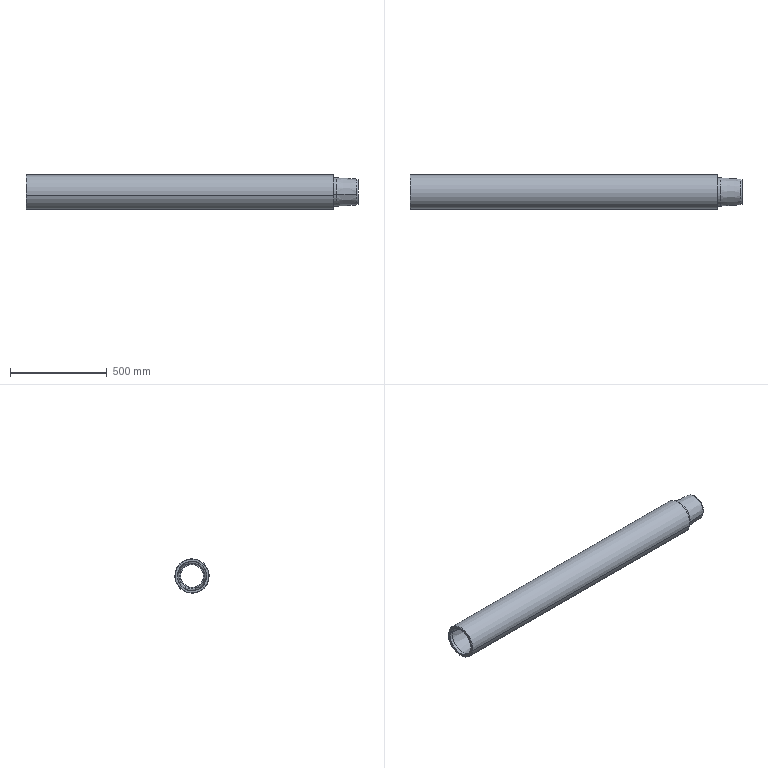Component | SolidWorks | 216OuterTube-1_OuterTube-1 | 1 solid | 31 faces | box 1717 x 178 x 178 mm | volume 22090156 mm3 | cone 16 | cylinder 10 | plane 5 | commonest cylinder face diameters 125.466 x2 150.01 x2 146.959 x2 118 x2 178 x2 | material Alloy Steel
build123d program:
from build123d import *


with BuildPart() as part:
    # Model → Revolve1 (revolve)
    with BuildSketch(Plane.XY, mode=Mode.PRIVATE) as revolve1_sk:
        Polygon((-900.264, 62.5), (-900.264, 59), (688.736, 59), (688.736, 62.484), (680.467, 67.258), (578.736, 73.48), (562.736, 73.48), (561.736, 74.48), (561.736, 89), (-1026.264, 89), (-1028.264, 87), (-1028.264, 75.886), (-1027.264, 74.886), (-1013.264, 74.029), (-1004.318, 68.864), align=None)
    revolve(revolve1_sk.sketch.rotate(Axis((0.1381, 0, 0), (1, 0, 0)), 180), axis=Axis((0.1381, 0, 0), (1, 0, 0)))

    # Sketch1 → Cut-Revolve1 (revolve, cut)
    with BuildSketch(Plane.XY, mode=Mode.PRIVATE) as cut_revolve1_sk:
        Polygon((-1027.943, 61), (-1027.943, 75.005), (-1011.709, 75.005), (-907.254, 68.616), (-901.264, 62.733), (-901.259, 62.733), (-901.259, 61), align=None)
    revolve(cut_revolve1_sk.sketch.rotate(Axis((-1032.943, 0, 0), (1, 0, 0)), 180), axis=Axis((-1032.943, 0, 0), (1, 0, 0)), mode=Mode.SUBTRACT)


solid = part.part

# Placed as in the assembly
solid = solid.moved(Location((1865.343, 0, 0), (0, 0, 0)))
STEP:
#1=CARTESIAN_POINT('',(37.956,2.431,0.4376));
#2=VERTEX_POINT('',#1);
#3=CARTESIAN_POINT('',(37.956,-2.431,-0.4376));
#4=VERTEX_POINT('',#3);
#5=CARTESIAN_POINT('',(37.956,-0.,0.));
#6=DIRECTION('',(-1.,-0.,0.));
#7=DIRECTION('',(0.,-0.9842,-0.1772));
#8=AXIS2_PLACEMENT_3D('',#5,#6,#7);
#9=CIRCLE('',#8,2.47);
#10=EDGE_CURVE('',#2,#4,#9,.T.);
#11=ORIENTED_EDGE('',*,*,#10,.F.);
#12=CARTESIAN_POINT('',(37.956,2.431,0.4376));
#13=VERTEX_POINT('',#12);
#14=CARTESIAN_POINT('',(32.772,2.431,0.4376));
#15=DIRECTION('',(-1.,-0.,0.));
#16=VECTOR('',#15,39.37);
#17=LINE('',#14,#16);
#18=EDGE_CURVE('',#2,#13,#17,.T.);
#19=ORIENTED_EDGE('',*,*,#18,.T.);
#20=CARTESIAN_POINT('',(37.956,-2.431,-0.4376));
#21=VERTEX_POINT('',#20);
#22=CARTESIAN_POINT('',(37.956,-0.,0.));
#23=DIRECTION('',(-1.,-0.,0.));
#24=DIRECTION('',(0.,-0.9842,-0.1772));
#25=AXIS2_PLACEMENT_3D('',#22,#23,#24);
#26=CIRCLE('',#25,2.47);
#27=EDGE_CURVE('',#13,#21,#26,.T.);
#28=ORIENTED_EDGE('',*,*,#27,.T.);
#29=CARTESIAN_POINT('',(32.772,-2.431,-0.4376));
#30=DIRECTION('',(-1.,-0.,0.));
#31=VECTOR('',#30,39.37);
#32=LINE('',#29,#31);
#33=EDGE_CURVE('',#4,#21,#32,.T.);
#34=ORIENTED_EDGE('',*,*,#33,.F.);
#35=EDGE_LOOP('',(#11,#19,#28,#34));
#36=FACE_OUTER_BOUND('',#35,.T.);
#37=CARTESIAN_POINT('',(32.772,-0.,0.));
#38=DIRECTION('',(-1.,-0.,0.));
#39=DIRECTION('',(0.,-0.9842,-0.1772));
#40=AXIS2_PLACEMENT_3D('',#37,#38,#39);
#41=CYLINDRICAL_SURFACE('',#40,2.47);
#42=ADVANCED_FACE('',(#36),#41,.F.);
#43=ORIENTED_EDGE('',*,*,#27,.F.);
#44=CARTESIAN_POINT('',(37.72,2.659,0.4786));
#45=VERTEX_POINT('',#44);
#46=CARTESIAN_POINT('',(37.956,2.431,0.4376));
#47=DIRECTION('',(-0.7134,0.6896,0.1242));
#48=VECTOR('',#47,39.37);
#49=LINE('',#46,#48);
#50=EDGE_CURVE('',#13,#45,#49,.T.);
#51=ORIENTED_EDGE('',*,*,#50,.T.);
#52=CARTESIAN_POINT('',(37.72,-2.659,-0.4786));
#53=VERTEX_POINT('',#52);
#54=CARTESIAN_POINT('',(37.72,-0.,0.));
#55=DIRECTION('',(-1.,-0.,0.));
#56=DIRECTION('',(0.,-0.9842,-0.1772));
#57=AXIS2_PLACEMENT_3D('',#54,#55,#56);
#58=CIRCLE('',#57,2.701);
#59=EDGE_CURVE('',#45,#53,#58,.T.);
#60=ORIENTED_EDGE('',*,*,#59,.T.);
#61=CARTESIAN_POINT('',(37.956,-2.431,-0.4376));
#62=DIRECTION('',(-0.7134,-0.6896,-0.1242));
#63=VECTOR('',#62,39.37);
#64=LINE('',#61,#63);
#65=EDGE_CURVE('',#21,#53,#64,.T.);
#66=ORIENTED_EDGE('',*,*,#65,.F.);
#67=EDGE_LOOP('',(#43,#51,#60,#66));
#68=FACE_OUTER_BOUND('',#67,.T.);
#69=CARTESIAN_POINT('',(37.956,-0.,0.));
#70=DIRECTION('',(-1.,-0.,0.));
#71=DIRECTION('',(0.,-0.9842,-0.1772));
#72=AXIS2_PLACEMENT_3D('',#69,#70,#71);
#73=CONICAL_SURFACE('',#72,2.47,0.7764);
#74=ADVANCED_FACE('',(#68),#73,.F.);
#75=ORIENTED_EDGE('',*,*,#59,.F.);
#76=CARTESIAN_POINT('',(33.608,2.906,0.5232));
#77=VERTEX_POINT('',#76);
#78=CARTESIAN_POINT('',(37.72,2.659,0.4786));
#79=DIRECTION('',(-0.9981,0.06008,0.01082));
#80=VECTOR('',#79,39.37);
#81=LINE('',#78,#80);
#82=EDGE_CURVE('',#45,#77,#81,.T.);
#83=ORIENTED_EDGE('',*,*,#82,.T.);
#84=CARTESIAN_POINT('',(33.608,-2.906,-0.5232));
#85=VERTEX_POINT('',#84);
#86=CARTESIAN_POINT('',(33.608,-0.,0.));
#87=DIRECTION('',(-1.,-0.,0.));
#88=DIRECTION('',(0.,-0.9842,-0.1772));
#89=AXIS2_PLACEMENT_3D('',#86,#87,#88);
#90=CIRCLE('',#89,2.953);
#91=EDGE_CURVE('',#77,#85,#90,.T.);
#92=ORIENTED_EDGE('',*,*,#91,.T.);
#93=CARTESIAN_POINT('',(37.72,-2.659,-0.4786));
#94=DIRECTION('',(-0.9981,-0.06008,-0.01082));
#95=VECTOR('',#94,39.37);
#96=LINE('',#93,#95);
#97=EDGE_CURVE('',#53,#85,#96,.T.);
#98=ORIENTED_EDGE('',*,*,#97,.F.);
#99=EDGE_LOOP('',(#75,#83,#92,#98));
#100=FACE_OUTER_BOUND('',#99,.T.);
#101=CARTESIAN_POINT('',(37.72,-0.,0.));
#102=DIRECTION('',(-1.,-0.,0.));
#103=DIRECTION('',(0.,-0.9842,-0.1772));
#104=AXIS2_PLACEMENT_3D('',#101,#102,#103);
#105=CONICAL_SURFACE('',#104,2.701,0.06109);
#106=ADVANCED_FACE('',(#100),#105,.F.);
#107=ORIENTED_EDGE('',*,*,#91,.F.);
#108=CARTESIAN_POINT('',(32.991,2.906,0.5232));
#109=VERTEX_POINT('',#108);
#110=CARTESIAN_POINT('',(32.772,2.906,0.5232));
#111=DIRECTION('',(-1.,-0.,0.));
#112=VECTOR('',#111,39.37);
#113=LINE('',#110,#112);
#114=EDGE_CURVE('',#77,#109,#113,.T.);
#115=ORIENTED_EDGE('',*,*,#114,.T.);
#116=CARTESIAN_POINT('',(32.991,-2.906,-0.5232));
#117=VERTEX_POINT('',#116);
#118=CARTESIAN_POINT('',(32.991,-0.,-0.));
#119=DIRECTION('',(-1.,-0.,0.));
#120=DIRECTION('',(0.,-0.9842,-0.1772));
#121=AXIS2_PLACEMENT_3D('',#118,#119,#120);
#122=CIRCLE('',#121,2.953);
#123=EDGE_CURVE('',#109,#117,#122,.T.);
#124=ORIENTED_EDGE('',*,*,#123,.T.);
#125=CARTESIAN_POINT('',(32.772,-2.906,-0.5232));
#126=DIRECTION('',(-1.,-0.,0.));
#127=VECTOR('',#126,39.37);
#128=LINE('',#125,#127);
#129=EDGE_CURVE('',#85,#117,#128,.T.);
#130=ORIENTED_EDGE('',*,*,#129,.F.);
#131=EDGE_LOOP('',(#107,#115,#124,#130));
#132=FACE_OUTER_BOUND('',#131,.T.);
#133=CARTESIAN_POINT('',(32.772,-0.,0.));
#134=DIRECTION('',(-1.,-0.,0.));
#135=DIRECTION('',(0.,-0.9842,-0.1772));
#136=AXIS2_PLACEMENT_3D('',#133,#134,#135);
#137=CYLINDRICAL_SURFACE('',#136,2.953);
#138=ADVANCED_FACE('',(#132),#137,.F.);
#139=CARTESIAN_POINT('',(95.594,-2.847,-0.5126));
#140=VERTEX_POINT('',#139);
#141=CARTESIAN_POINT('',(95.594,2.847,0.5126));
#142=VERTEX_POINT('',#141);
#143=CARTESIAN_POINT('',(95.594,-0.,-0.));
#144=DIRECTION('',(-1.,-0.,0.));
#145=DIRECTION('',(0.,-0.9842,-0.1772));
#146=AXIS2_PLACEMENT_3D('',#143,#144,#145);
#147=CIRCLE('',#146,2.893);
#148=EDGE_CURVE('',#140,#142,#147,.T.);
#149=ORIENTED_EDGE('',*,*,#148,.T.);
#150=CARTESIAN_POINT('',(95.554,2.886,0.5195));
#151=VERTEX_POINT('',#150);
#152=CARTESIAN_POINT('',(95.554,2.886,0.5195));
#153=DIRECTION('',(-0.7071,0.6959,0.1253));
#154=VECTOR('',#153,39.37);
#155=LINE('',#152,#154);
#156=EDGE_CURVE('',#142,#151,#155,.T.);
#157=ORIENTED_EDGE('',*,*,#156,.T.);
#158=CARTESIAN_POINT('',(95.554,-2.886,-0.5195));
#159=VERTEX_POINT('',#158);
#160=CARTESIAN_POINT('',(95.554,-0.,-0.));
#161=DIRECTION('',(-1.,-0.,0.));
#162=DIRECTION('',(0.,-0.9842,-0.1772));
#163=AXIS2_PLACEMENT_3D('',#160,#161,#162);
#164=CIRCLE('',#163,2.932);
#165=EDGE_CURVE('',#159,#151,#164,.T.);
#166=ORIENTED_EDGE('',*,*,#165,.F.);
#167=CARTESIAN_POINT('',(95.554,-2.886,-0.5195));
#168=DIRECTION('',(-0.7071,-0.6959,-0.1253));
#169=VECTOR('',#168,39.37);
#170=LINE('',#167,#169);
#171=EDGE_CURVE('',#140,#159,#170,.T.);
#172=ORIENTED_EDGE('',*,*,#171,.F.);
#173=EDGE_LOOP('',(#149,#157,#166,#172));
#174=FACE_OUTER_BOUND('',#173,.T.);
#175=CARTESIAN_POINT('',(95.554,-0.,-0.));
#176=DIRECTION('',(-1.,-0.,0.));
#177=DIRECTION('',(0.,-0.9842,-0.1772));
#178=AXIS2_PLACEMENT_3D('',#175,#176,#177);
#179=CONICAL_SURFACE('',#178,2.932,0.7854);
#180=ADVANCED_FACE('',(#174),#179,.T.);
#181=CARTESIAN_POINT('',(96.224,-2.847,-0.5126));
#182=VERTEX_POINT('',#181);
#183=CARTESIAN_POINT('',(96.224,2.847,0.5126));
#184=VERTEX_POINT('',#183);
#185=CARTESIAN_POINT('',(96.224,-0.,-0.));
#186=DIRECTION('',(-1.,-0.,0.));
#187=DIRECTION('',(0.,-0.9842,-0.1772));
#188=AXIS2_PLACEMENT_3D('',#185,#186,#187);
#189=CIRCLE('',#188,2.893);
#190=EDGE_CURVE('',#182,#184,#189,.T.);
#191=ORIENTED_EDGE('',*,*,#190,.T.);
#192=CARTESIAN_POINT('',(73.444,2.847,0.5126));
#193=DIRECTION('',(-1.,-0.,0.));
#194=VECTOR('',#193,39.37);
#195=LINE('',#192,#194);
#196=EDGE_CURVE('',#184,#142,#195,.T.);
#197=ORIENTED_EDGE('',*,*,#196,.T.);
#198=ORIENTED_EDGE('',*,*,#148,.F.);
#199=CARTESIAN_POINT('',(73.444,-2.847,-0.5126));
#200=DIRECTION('',(-1.,-0.,0.));
#201=VECTOR('',#200,39.37);
#202=LINE('',#199,#201);
#203=EDGE_CURVE('',#182,#140,#202,.T.);
#204=ORIENTED_EDGE('',*,*,#203,.F.);
#205=EDGE_LOOP('',(#191,#197,#198,#204));
#206=FACE_OUTER_BOUND('',#205,.T.);
#207=CARTESIAN_POINT('',(73.444,-0.,-0.));
#208=DIRECTION('',(-1.,-0.,0.));
#209=DIRECTION('',(0.,-0.9842,-0.1772));
#210=AXIS2_PLACEMENT_3D('',#207,#208,#209);
#211=CYLINDRICAL_SURFACE('',#210,2.893);
#212=ADVANCED_FACE('',(#206),#211,.T.);
#213=CARTESIAN_POINT('',(100.229,-2.606,-0.4692));
#214=VERTEX_POINT('',#213);
#215=CARTESIAN_POINT('',(100.229,2.606,0.4692));
#216=VERTEX_POINT('',#215);
#217=CARTESIAN_POINT('',(100.229,-0.,-0.));
#218=DIRECTION('',(-1.,-0.,0.));
#219=DIRECTION('',(0.,-0.9842,-0.1772));
#220=AXIS2_PLACEMENT_3D('',#217,#218,#219);
#221=CIRCLE('',#220,2.648);
#222=EDGE_CURVE('',#214,#216,#221,.T.);
#223=ORIENTED_EDGE('',*,*,#222,.T.);
#224=CARTESIAN_POINT('',(96.224,2.847,0.5126));
#225=DIRECTION('',(-0.9981,0.06008,0.01082));
#226=VECTOR('',#225,39.37);
#227=LINE('',#224,#226);
#228=EDGE_CURVE('',#216,#184,#227,.T.);
#229=ORIENTED_EDGE('',*,*,#228,.T.);
#230=ORIENTED_EDGE('',*,*,#190,.F.);
#231=CARTESIAN_POINT('',(96.224,-2.847,-0.5126));
#232=DIRECTION('',(-0.9981,-0.06008,-0.01082));
#233=VECTOR('',#232,39.37);
#234=LINE('',#231,#233);
#235=EDGE_CURVE('',#214,#182,#234,.T.);
#236=ORIENTED_EDGE('',*,*,#235,.F.);
#237=EDGE_LOOP('',(#223,#229,#230,#236));
#238=FACE_OUTER_BOUND('',#237,.T.);
#239=CARTESIAN_POINT('',(96.224,-0.,-0.));
#240=DIRECTION('',(-1.,-0.,0.));
#241=DIRECTION('',(0.,-0.9842,-0.1772));
#242=AXIS2_PLACEMENT_3D('',#239,#240,#241);
#243=CONICAL_SURFACE('',#242,2.893,0.06109);
#244=ADVANCED_FACE('',(#238),#243,.T.);
#245=CARTESIAN_POINT('',(100.554,-2.421,-0.4359));
#246=VERTEX_POINT('',#245);
#247=CARTESIAN_POINT('',(100.554,2.421,0.4359));
#248=VERTEX_POINT('',#247);
#249=CARTESIAN_POINT('',(100.554,-0.,-0.));
#250=DIRECTION('',(-1.,-0.,0.));
#251=DIRECTION('',(0.,-0.9842,-0.1772));
#252=AXIS2_PLACEMENT_3D('',#249,#250,#251);
#253=CIRCLE('',#252,2.46);
#254=EDGE_CURVE('',#246,#248,#253,.T.);
#255=ORIENTED_EDGE('',*,*,#254,.T.);
#256=CARTESIAN_POINT('',(100.229,2.606,0.4692));
#257=DIRECTION('',(-0.866,0.4921,0.08859));
#258=VECTOR('',#257,39.37);
#259=LINE('',#256,#258);
#260=EDGE_CURVE('',#248,#216,#259,.T.);
#261=ORIENTED_EDGE('',*,*,#260,.T.);
#262=ORIENTED_EDGE('',*,*,#222,.F.);
#263=CARTESIAN_POINT('',(100.229,-2.606,-0.4692));
#264=DIRECTION('',(-0.866,-0.4921,-0.08859));
#265=VECTOR('',#264,39.37);
#266=LINE('',#263,#265);
#267=EDGE_CURVE('',#246,#214,#266,.T.);
#268=ORIENTED_EDGE('',*,*,#267,.F.);
#269=EDGE_LOOP('',(#255,#261,#262,#268));
#270=FACE_OUTER_BOUND('',#269,.T.);
#271=CARTESIAN_POINT('',(100.229,-0.,-0.));
#272=DIRECTION('',(-1.,-0.,0.));
#273=DIRECTION('',(0.,-0.9842,-0.1772));
#274=AXIS2_PLACEMENT_3D('',#271,#272,#273);
#275=CONICAL_SURFACE('',#274,2.648,0.5236);
#276=ADVANCED_FACE('',(#270),#275,.T.);
#277=CARTESIAN_POINT('',(100.554,2.286,0.4116));
#278=VERTEX_POINT('',#277);
#279=CARTESIAN_POINT('',(100.554,-2.286,-0.4116));
#280=VERTEX_POINT('',#279);
#281=CARTESIAN_POINT('',(100.554,-0.,-0.));
#282=DIRECTION('',(-1.,-0.,0.));
#283=DIRECTION('',(0.,-0.9842,-0.1772));
#284=AXIS2_PLACEMENT_3D('',#281,#282,#283);
#285=CIRCLE('',#284,2.323);
#286=EDGE_CURVE('',#278,#280,#285,.T.);
#287=ORIENTED_EDGE('',*,*,#286,.F.);
#288=CARTESIAN_POINT('',(37.995,2.286,0.4116));
#289=VERTEX_POINT('',#288);
#290=CARTESIAN_POINT('',(73.444,2.286,0.4116));
#291=DIRECTION('',(-1.,-0.,0.));
#292=VECTOR('',#291,39.37);
#293=LINE('',#290,#292);
#294=EDGE_CURVE('',#278,#289,#293,.T.);
#295=ORIENTED_EDGE('',*,*,#294,.T.);
#296=CARTESIAN_POINT('',(37.995,-2.286,-0.4116));
#297=VERTEX_POINT('',#296);
#298=CARTESIAN_POINT('',(37.995,-0.,-0.));
#299=DIRECTION('',(-1.,-0.,0.));
#300=DIRECTION('',(0.,-0.9842,-0.1772));
#301=AXIS2_PLACEMENT_3D('',#298,#299,#300);
#302=CIRCLE('',#301,2.323);
#303=EDGE_CURVE('',#289,#297,#302,.T.);
#304=ORIENTED_EDGE('',*,*,#303,.T.);
#305=CARTESIAN_POINT('',(73.444,-2.286,-0.4116));
#306=DIRECTION('',(-1.,-0.,0.));
#307=VECTOR('',#306,39.37);
#308=LINE('',#305,#307);
#309=EDGE_CURVE('',#280,#297,#308,.T.);
#310=ORIENTED_EDGE('',*,*,#309,.F.);
#311=EDGE_LOOP('',(#287,#295,#304,#310));
#312=FACE_OUTER_BOUND('',#311,.T.);
#313=CARTESIAN_POINT('',(73.444,-0.,-0.));
#314=DIRECTION('',(-1.,-0.,0.));
#315=DIRECTION('',(0.,-0.9842,-0.1772));
#316=AXIS2_PLACEMENT_3D('',#313,#314,#315);
#317=CYLINDRICAL_SURFACE('',#316,2.323);
#318=ADVANCED_FACE('',(#312),#317,.F.);
#319=CARTESIAN_POINT('',(32.956,-3.371,-0.6069));
#320=VERTEX_POINT('',#319);
#321=CARTESIAN_POINT('',(32.956,3.371,0.6069));
#322=VERTEX_POINT('',#321);
#323=CARTESIAN_POINT('',(32.956,-0.,-0.));
#324=DIRECTION('',(-1.,-0.,0.));
#325=DIRECTION('',(0.,-0.9842,-0.1772));
#326=AXIS2_PLACEMENT_3D('',#323,#324,#325);
#327=CIRCLE('',#326,3.425);
#328=EDGE_CURVE('',#320,#322,#327,.T.);
#329=ORIENTED_EDGE('',*,*,#328,.F.);
#330=CARTESIAN_POINT('',(33.035,-3.448,-0.6208));
#331=VERTEX_POINT('',#330);
#332=CARTESIAN_POINT('',(33.035,-3.448,-0.6208));
#333=DIRECTION('',(0.7071,-0.6959,-0.1253));
#334=VECTOR('',#333,39.37);
#335=LINE('',#332,#334);
#336=EDGE_CURVE('',#320,#331,#335,.T.);
#337=ORIENTED_EDGE('',*,*,#336,.T.);
#338=CARTESIAN_POINT('',(33.035,3.448,0.6208));
#339=VERTEX_POINT('',#338);
#340=CARTESIAN_POINT('',(33.035,-0.,-0.));
#341=DIRECTION('',(-1.,-0.,0.));
#342=DIRECTION('',(0.,-0.9842,-0.1772));
#343=AXIS2_PLACEMENT_3D('',#340,#341,#342);
#344=CIRCLE('',#343,3.504);
#345=EDGE_CURVE('',#331,#339,#344,.T.);
#346=ORIENTED_EDGE('',*,*,#345,.T.);
#347=CARTESIAN_POINT('',(33.035,3.448,0.6208));
#348=DIRECTION('',(0.7071,0.6959,0.1253));
#349=VECTOR('',#348,39.37);
#350=LINE('',#347,#349);
#351=EDGE_CURVE('',#322,#339,#350,.T.);
#352=ORIENTED_EDGE('',*,*,#351,.F.);
#353=EDGE_LOOP('',(#329,#337,#346,#352));
#354=FACE_OUTER_BOUND('',#353,.T.);
#355=CARTESIAN_POINT('',(33.035,-0.,-0.));
#356=DIRECTION('',(1.,0.,-0.));
#357=DIRECTION('',(0.,0.9842,0.1772));
#358=AXIS2_PLACEMENT_3D('',#355,#356,#357);
#359=CONICAL_SURFACE('',#358,3.504,0.7854);
#360=ADVANCED_FACE('',(#354),#359,.T.);
#361=CARTESIAN_POINT('',(95.554,-3.448,-0.6208));
#362=VERTEX_POINT('',#361);
#363=CARTESIAN_POINT('',(95.554,3.448,0.6208));
#364=VERTEX_POINT('',#363);
#365=CARTESIAN_POINT('',(95.554,-0.,-0.));
#366=DIRECTION('',(-1.,-0.,0.));
#367=DIRECTION('',(0.,-0.9842,-0.1772));
#368=AXIS2_PLACEMENT_3D('',#365,#366,#367);
#369=CIRCLE('',#368,3.504);
#370=EDGE_CURVE('',#362,#364,#369,.T.);
#371=ORIENTED_EDGE('',*,*,#370,.T.);
#372=CARTESIAN_POINT('',(73.444,3.448,0.6208));
#373=DIRECTION('',(-1.,-0.,0.));
#374=VECTOR('',#373,39.37);
#375=LINE('',#372,#374);
#376=EDGE_CURVE('',#364,#339,#375,.T.);
#377=ORIENTED_EDGE('',*,*,#376,.T.);
#378=ORIENTED_EDGE('',*,*,#345,.F.);
#379=CARTESIAN_POINT('',(73.444,-3.448,-0.6208));
#380=DIRECTION('',(-1.,-0.,0.));
#381=VECTOR('',#380,39.37);
#382=LINE('',#379,#381);
#383=EDGE_CURVE('',#362,#331,#382,.T.);
#384=ORIENTED_EDGE('',*,*,#383,.F.);
#385=EDGE_LOOP('',(#371,#377,#378,#384));
#386=FACE_OUTER_BOUND('',#385,.T.);
#387=CARTESIAN_POINT('',(73.444,-0.,-0.));
#388=DIRECTION('',(-1.,-0.,0.));
#389=DIRECTION('',(0.,-0.9842,-0.1772));
#390=AXIS2_PLACEMENT_3D('',#387,#388,#389);
#391=CYLINDRICAL_SURFACE('',#390,3.504);
#392=ADVANCED_FACE('',(#386),#391,.T.);
#393=CARTESIAN_POINT('',(37.995,2.422,0.436));
#394=VERTEX_POINT('',#393);
#395=CARTESIAN_POINT('',(37.995,-2.422,-0.436));
#396=VERTEX_POINT('',#395);
#397=CARTESIAN_POINT('',(37.995,-0.,-0.));
#398=DIRECTION('',(-1.,-0.,0.));
#399=DIRECTION('',(0.,-0.9842,-0.1772));
#400=AXIS2_PLACEMENT_3D('',#397,#398,#399);
#401=CIRCLE('',#400,2.461);
#402=EDGE_CURVE('',#394,#396,#401,.T.);
#403=ORIENTED_EDGE('',*,*,#402,.F.);
#404=CARTESIAN_POINT('',(37.956,2.424,0.4364));
#405=VERTEX_POINT('',#404);
#406=CARTESIAN_POINT('',(33.899,2.668,0.4804));
#407=DIRECTION('',(-0.9981,0.06008,0.01082));
#408=VECTOR('',#407,39.37);
#409=LINE('',#406,#408);
#410=EDGE_CURVE('',#394,#405,#409,.T.);
#411=ORIENTED_EDGE('',*,*,#410,.T.);
#412=CARTESIAN_POINT('',(37.956,-2.424,-0.4364));
#413=VERTEX_POINT('',#412);
#414=CARTESIAN_POINT('',(37.956,-0.,-0.));
#415=DIRECTION('',(1.,0.,-0.));
#416=DIRECTION('',(0.,-0.9842,-0.1772));
#417=AXIS2_PLACEMENT_3D('',#414,#415,#416);
#418=CIRCLE('',#417,2.463);
#419=EDGE_CURVE('',#413,#405,#418,.T.);
#420=ORIENTED_EDGE('',*,*,#419,.F.);
#421=CARTESIAN_POINT('',(33.899,-2.668,-0.4804));
#422=DIRECTION('',(-0.9981,-0.06008,-0.01082));
#423=VECTOR('',#422,39.37);
#424=LINE('',#421,#423);
#425=EDGE_CURVE('',#396,#413,#424,.T.);
#426=ORIENTED_EDGE('',*,*,#425,.F.);
#427=EDGE_LOOP('',(#403,#411,#420,#426));
#428=FACE_OUTER_BOUND('',#427,.T.);
#429=CARTESIAN_POINT('',(33.899,-0.,-0.));
#430=DIRECTION('',(-1.,-0.,0.));
#431=DIRECTION('',(0.,-0.9842,-0.1772));
#432=AXIS2_PLACEMENT_3D('',#429,#430,#431);
#433=CONICAL_SURFACE('',#432,2.711,0.06109);
#434=ADVANCED_FACE('',(#428),#433,.F.);
#435=ORIENTED_EDGE('',*,*,#123,.F.);
#436=CARTESIAN_POINT('',(32.956,2.94,0.5294));
#437=VERTEX_POINT('',#436);
#438=CARTESIAN_POINT('',(32.956,2.94,0.5294));
#439=DIRECTION('',(-0.7071,0.6959,0.1253));
#440=VECTOR('',#439,39.37);
#441=LINE('',#438,#440);
#442=EDGE_CURVE('',#109,#437,#441,.T.);
#443=ORIENTED_EDGE('',*,*,#442,.T.);
#444=CARTESIAN_POINT('',(32.956,-2.94,-0.5294));
#445=VERTEX_POINT('',#444);
#446=CARTESIAN_POINT('',(32.956,-0.,-0.));
#447=DIRECTION('',(-1.,-0.,0.));
#448=DIRECTION('',(0.,-0.9842,-0.1772));
#449=AXIS2_PLACEMENT_3D('',#446,#447,#448);
#450=CIRCLE('',#449,2.988);
#451=EDGE_CURVE('',#437,#445,#450,.T.);
#452=ORIENTED_EDGE('',*,*,#451,.T.);
#453=CARTESIAN_POINT('',(32.956,-2.94,-0.5294));
#454=DIRECTION('',(-0.7071,-0.6959,-0.1253));
#455=VECTOR('',#454,39.37);
#456=LINE('',#453,#455);
#457=EDGE_CURVE('',#117,#445,#456,.T.);
#458=ORIENTED_EDGE('',*,*,#457,.F.);
#459=EDGE_LOOP('',(#435,#443,#452,#458));
#460=FACE_OUTER_BOUND('',#459,.T.);
#461=CARTESIAN_POINT('',(32.956,-0.,-0.));
#462=DIRECTION('',(-1.,-0.,0.));
#463=DIRECTION('',(0.,-0.9842,-0.1772));
#464=AXIS2_PLACEMENT_3D('',#461,#462,#463);
#465=CONICAL_SURFACE('',#464,2.988,0.7854);
#466=ADVANCED_FACE('',(#460),#465,.F.);
#467=ORIENTED_EDGE('',*,*,#442,.F.);
#468=CARTESIAN_POINT('',(32.991,-0.,-0.));
#469=DIRECTION('',(-1.,-0.,0.));
#470=DIRECTION('',(0.,-0.9842,-0.1772));
#471=AXIS2_PLACEMENT_3D('',#468,#469,#470);
#472=CIRCLE('',#471,2.953);
#473=EDGE_CURVE('',#117,#109,#472,.T.);
#474=ORIENTED_EDGE('',*,*,#473,.F.);
#475=ORIENTED_EDGE('',*,*,#457,.T.);
#476=CARTESIAN_POINT('',(32.956,-0.,-0.));
#477=DIRECTION('',(-1.,-0.,0.));
#478=DIRECTION('',(0.,-0.9842,-0.1772));
#479=AXIS2_PLACEMENT_3D('',#476,#477,#478);
#480=CIRCLE('',#479,2.988);
#481=EDGE_CURVE('',#445,#437,#480,.T.);
#482=ORIENTED_EDGE('',*,*,#481,.T.);
#483=EDGE_LOOP('',(#467,#474,#475,#482));
#484=FACE_OUTER_BOUND('',#483,.T.);
#485=CARTESIAN_POINT('',(32.956,-0.,-0.));
#486=DIRECTION('',(-1.,-0.,0.));
#487=DIRECTION('',(0.,-0.9842,-0.1772));
#488=AXIS2_PLACEMENT_3D('',#485,#486,#487);
#489=CONICAL_SURFACE('',#488,2.988,0.7854);
#490=ADVANCED_FACE('',(#484),#489,.F.);
#491=ORIENTED_EDGE('',*,*,#410,.F.);
#492=CARTESIAN_POINT('',(37.995,-0.,-0.));
#493=DIRECTION('',(-1.,-0.,0.));
#494=DIRECTION('',(0.,-0.9842,-0.1772));
#495=AXIS2_PLACEMENT_3D('',#492,#493,#494);
#496=CIRCLE('',#495,2.461);
#497=EDGE_CURVE('',#396,#394,#496,.T.);
#498=ORIENTED_EDGE('',*,*,#497,.F.);
#499=ORIENTED_EDGE('',*,*,#425,.T.);
#500=CARTESIAN_POINT('',(37.956,-0.,-0.));
#501=DIRECTION('',(1.,0.,-0.));
#502=DIRECTION('',(0.,-0.9842,-0.1772));
#503=AXIS2_PLACEMENT_3D('',#500,#501,#502);
#504=CIRCLE('',#503,2.463);
#505=EDGE_CURVE('',#405,#413,#504,.T.);
#506=ORIENTED_EDGE('',*,*,#505,.F.);
#507=EDGE_LOOP('',(#491,#498,#499,#506));
#508=FACE_OUTER_BOUND('',#507,.T.);
#509=CARTESIAN_POINT('',(33.899,-0.,-0.));
#510=DIRECTION('',(-1.,-0.,0.));
#511=DIRECTION('',(0.,-0.9842,-0.1772));
#512=AXIS2_PLACEMENT_3D('',#509,#510,#511);
#513=CONICAL_SURFACE('',#512,2.711,0.06109);
#514=ADVANCED_FACE('',(#508),#513,.F.);
#515=ORIENTED_EDGE('',*,*,#165,.T.);
#516=CARTESIAN_POINT('',(95.554,-0.,-0.));
#517=DIRECTION('',(-1.,-0.,0.));
#518=DIRECTION('',(0.,-0.9842,-0.1772));
#519=AXIS2_PLACEMENT_3D('',#516,#517,#518);
#520=CIRCLE('',#519,2.932);
#521=EDGE_CURVE('',#151,#159,#520,.T.);
#522=ORIENTED_EDGE('',*,*,#521,.T.);
#523=EDGE_LOOP('',(#515,#522));
#524=FACE_BOUND('',#523,.T.);
#525=ORIENTED_EDGE('',*,*,#370,.F.);
#526=CARTESIAN_POINT('',(95.554,-0.,-0.));
#527=DIRECTION('',(-1.,-0.,0.));
#528=DIRECTION('',(0.,-0.9842,-0.1772));
#529=AXIS2_PLACEMENT_3D('',#526,#527,#528);
#530=CIRCLE('',#529,3.504);
#531=EDGE_CURVE('',#364,#362,#530,.T.);
#532=ORIENTED_EDGE('',*,*,#531,.F.);
#533=EDGE_LOOP('',(#525,#532));
#534=FACE_OUTER_BOUND('',#533,.T.);
#535=CARTESIAN_POINT('',(95.554,-0.,-0.));
#536=DIRECTION('',(1.,0.,-0.));
#537=DIRECTION('',(-0.,0.9842,0.1772));
#538=AXIS2_PLACEMENT_3D('',#535,#536,#537);
#539=PLANE('',#538);
#540=ADVANCED_FACE('',(#524,#534),#539,.T.);
#541=ORIENTED_EDGE('',*,*,#376,.F.);
#542=ORIENTED_EDGE('',*,*,#531,.T.);
#543=ORIENTED_EDGE('',*,*,#383,.T.);
#544=CARTESIAN_POINT('',(33.035,-0.,-0.));
#545=DIRECTION('',(-1.,-0.,0.));
#546=DIRECTION('',(0.,-0.9842,-0.1772));
#547=AXIS2_PLACEMENT_3D('',#544,#545,#546);
#548=CIRCLE('',#547,3.504);
#549=EDGE_CURVE('',#339,#331,#548,.T.);
#550=ORIENTED_EDGE('',*,*,#549,.F.);
#551=EDGE_LOOP('',(#541,#542,#543,#550));
#552=FACE_OUTER_BOUND('',#551,.T.);
#553=CARTESIAN_POINT('',(73.444,-0.,-0.));
#554=DIRECTION('',(-1.,-0.,0.));
#555=DIRECTION('',(0.,-0.9842,-0.1772));
#556=AXIS2_PLACEMENT_3D('',#553,#554,#555);
#557=CYLINDRICAL_SURFACE('',#556,3.504);
#558=ADVANCED_FACE('',(#552),#557,.T.);
#559=ORIENTED_EDGE('',*,*,#336,.F.);
#560=CARTESIAN_POINT('',(32.956,-0.,-0.));
#561=DIRECTION('',(-1.,-0.,0.));
#562=DIRECTION('',(0.,-0.9842,-0.1772));
#563=AXIS2_PLACEMENT_3D('',#560,#561,#562);
#564=CIRCLE('',#563,3.425);
#565=EDGE_CURVE('',#322,#320,#564,.T.);
#566=ORIENTED_EDGE('',*,*,#565,.F.);
#567=ORIENTED_EDGE('',*,*,#351,.T.);
#568=ORIENTED_EDGE('',*,*,#549,.T.);
#569=EDGE_LOOP('',(#559,#566,#567,#568));
#570=FACE_OUTER_BOUND('',#569,.T.);
#571=CARTESIAN_POINT('',(33.035,-0.,-0.));
#572=DIRECTION('',(1.,0.,-0.));
#573=DIRECTION('',(0.,0.9842,0.1772));
#574=AXIS2_PLACEMENT_3D('',#571,#572,#573);
#575=CONICAL_SURFACE('',#574,3.504,0.7854);
#576=ADVANCED_FACE('',(#570),#575,.T.);
#577=ORIENTED_EDGE('',*,*,#481,.F.);
#578=ORIENTED_EDGE('',*,*,#451,.F.);
#579=EDGE_LOOP('',(#577,#578));
#580=FACE_BOUND('',#579,.T.);
#581=ORIENTED_EDGE('',*,*,#565,.T.);
#582=ORIENTED_EDGE('',*,*,#328,.T.);
#583=EDGE_LOOP('',(#581,#582));
#584=FACE_OUTER_BOUND('',#583,.T.);
#585=CARTESIAN_POINT('',(32.956,-0.,0.));
#586=DIRECTION('',(1.,0.,-0.));
#587=DIRECTION('',(-0.,0.9842,0.1772));
#588=AXIS2_PLACEMENT_3D('',#585,#586,#587);
#589=PLANE('',#588);
#590=ADVANCED_FACE('',(#580,#584),#589,.F.);
#591=CARTESIAN_POINT('',(37.995,-0.,-0.));
#592=DIRECTION('',(-1.,-0.,0.));
#593=DIRECTION('',(0.,-0.9842,-0.1772));
#594=AXIS2_PLACEMENT_3D('',#591,#592,#593);
#595=CIRCLE('',#594,2.323);
#596=EDGE_CURVE('',#297,#289,#595,.T.);
#597=ORIENTED_EDGE('',*,*,#596,.F.);
#598=ORIENTED_EDGE('',*,*,#303,.F.);
#599=EDGE_LOOP('',(#597,#598));
#600=FACE_BOUND('',#599,.T.);
#601=ORIENTED_EDGE('',*,*,#497,.T.);
#602=ORIENTED_EDGE('',*,*,#402,.T.);
#603=EDGE_LOOP('',(#601,#602));
#604=FACE_OUTER_BOUND('',#603,.T.);
#605=CARTESIAN_POINT('',(37.995,-0.,0.));
#606=DIRECTION('',(1.,0.,-0.));
#607=DIRECTION('',(-0.,0.9842,0.1772));
#608=AXIS2_PLACEMENT_3D('',#605,#606,#607);
#609=PLANE('',#608);
#610=ADVANCED_FACE('',(#600,#604),#609,.F.);
#611=ORIENTED_EDGE('',*,*,#294,.F.);
#612=CARTESIAN_POINT('',(100.554,-0.,-0.));
#613=DIRECTION('',(-1.,-0.,0.));
#614=DIRECTION('',(0.,-0.9842,-0.1772));
#615=AXIS2_PLACEMENT_3D('',#612,#613,#614);
#616=CIRCLE('',#615,2.323);
#617=EDGE_CURVE('',#280,#278,#616,.T.);
#618=ORIENTED_EDGE('',*,*,#617,.F.);
#619=ORIENTED_EDGE('',*,*,#309,.T.);
#620=ORIENTED_EDGE('',*,*,#596,.T.);
#621=EDGE_LOOP('',(#611,#618,#619,#620));
#622=FACE_OUTER_BOUND('',#621,.T.);
#623=CARTESIAN_POINT('',(73.444,-0.,-0.));
#624=DIRECTION('',(-1.,-0.,0.));
#625=DIRECTION('',(0.,-0.9842,-0.1772));
#626=AXIS2_PLACEMENT_3D('',#623,#624,#625);
#627=CYLINDRICAL_SURFACE('',#626,2.323);
#628=ADVANCED_FACE('',(#622),#627,.F.);
#629=ORIENTED_EDGE('',*,*,#617,.T.);
#630=ORIENTED_EDGE('',*,*,#286,.T.);
#631=EDGE_LOOP('',(#629,#630));
#632=FACE_BOUND('',#631,.T.);
#633=ORIENTED_EDGE('',*,*,#254,.F.);
#634=CARTESIAN_POINT('',(100.554,-0.,-0.));
#635=DIRECTION('',(-1.,-0.,0.));
#636=DIRECTION('',(0.,-0.9842,-0.1772));
#637=AXIS2_PLACEMENT_3D('',#634,#635,#636);
#638=CIRCLE('',#637,2.46);
#639=EDGE_CURVE('',#248,#246,#638,.T.);
#640=ORIENTED_EDGE('',*,*,#639,.F.);
#641=EDGE_LOOP('',(#633,#640));
#642=FACE_OUTER_BOUND('',#641,.T.);
#643=CARTESIAN_POINT('',(100.554,-0.,-0.));
#644=DIRECTION('',(1.,0.,-0.));
#645=DIRECTION('',(-0.,0.9842,0.1772));
#646=AXIS2_PLACEMENT_3D('',#643,#644,#645);
#647=PLANE('',#646);
#648=ADVANCED_FACE('',(#632,#642),#647,.T.);
#649=ORIENTED_EDGE('',*,*,#260,.F.);
#650=ORIENTED_EDGE('',*,*,#639,.T.);
#651=ORIENTED_EDGE('',*,*,#267,.T.);
#652=CARTESIAN_POINT('',(100.229,-0.,-0.));
#653=DIRECTION('',(-1.,-0.,0.));
#654=DIRECTION('',(0.,-0.9842,-0.1772));
#655=AXIS2_PLACEMENT_3D('',#652,#653,#654);
#656=CIRCLE('',#655,2.648);
#657=EDGE_CURVE('',#216,#214,#656,.T.);
#658=ORIENTED_EDGE('',*,*,#657,.F.);
#659=EDGE_LOOP('',(#649,#650,#651,#658));
#660=FACE_OUTER_BOUND('',#659,.T.);
#661=CARTESIAN_POINT('',(100.229,-0.,-0.));
#662=DIRECTION('',(-1.,-0.,0.));
#663=DIRECTION('',(0.,-0.9842,-0.1772));
#664=AXIS2_PLACEMENT_3D('',#661,#662,#663);
#665=CONICAL_SURFACE('',#664,2.648,0.5236);
#666=ADVANCED_FACE('',(#660),#665,.T.);
#667=ORIENTED_EDGE('',*,*,#228,.F.);
#668=ORIENTED_EDGE('',*,*,#657,.T.);
#669=ORIENTED_EDGE('',*,*,#235,.T.);
#670=CARTESIAN_POINT('',(96.224,-0.,-0.));
#671=DIRECTION('',(-1.,-0.,0.));
#672=DIRECTION('',(0.,-0.9842,-0.1772));
#673=AXIS2_PLACEMENT_3D('',#670,#671,#672);
#674=CIRCLE('',#673,2.893);
#675=EDGE_CURVE('',#184,#182,#674,.T.);
#676=ORIENTED_EDGE('',*,*,#675,.F.);
#677=EDGE_LOOP('',(#667,#668,#669,#676));
#678=FACE_OUTER_BOUND('',#677,.T.);
#679=CARTESIAN_POINT('',(96.224,-0.,-0.));
#680=DIRECTION('',(-1.,-0.,0.));
#681=DIRECTION('',(0.,-0.9842,-0.1772));
#682=AXIS2_PLACEMENT_3D('',#679,#680,#681);
#683=CONICAL_SURFACE('',#682,2.893,0.06109);
#684=ADVANCED_FACE('',(#678),#683,.T.);
#685=ORIENTED_EDGE('',*,*,#196,.F.);
#686=ORIENTED_EDGE('',*,*,#675,.T.);
#687=ORIENTED_EDGE('',*,*,#203,.T.);
#688=CARTESIAN_POINT('',(95.594,-0.,-0.));
#689=DIRECTION('',(-1.,-0.,0.));
#690=DIRECTION('',(0.,-0.9842,-0.1772));
#691=AXIS2_PLACEMENT_3D('',#688,#689,#690);
#692=CIRCLE('',#691,2.893);
#693=EDGE_CURVE('',#142,#140,#692,.T.);
#694=ORIENTED_EDGE('',*,*,#693,.F.);
#695=EDGE_LOOP('',(#685,#686,#687,#694));
#696=FACE_OUTER_BOUND('',#695,.T.);
#697=CARTESIAN_POINT('',(73.444,-0.,-0.));
#698=DIRECTION('',(-1.,-0.,0.));
#699=DIRECTION('',(0.,-0.9842,-0.1772));
#700=AXIS2_PLACEMENT_3D('',#697,#698,#699);
#701=CYLINDRICAL_SURFACE('',#700,2.893);
#702=ADVANCED_FACE('',(#696),#701,.T.);
#703=ORIENTED_EDGE('',*,*,#156,.F.);
#704=ORIENTED_EDGE('',*,*,#693,.T.);
#705=ORIENTED_EDGE('',*,*,#171,.T.);
#706=ORIENTED_EDGE('',*,*,#521,.F.);
#707=EDGE_LOOP('',(#703,#704,#705,#706));
#708=FACE_OUTER_BOUND('',#707,.T.);
#709=CARTESIAN_POINT('',(95.554,-0.,-0.));
#710=DIRECTION('',(-1.,-0.,0.));
#711=DIRECTION('',(0.,-0.9842,-0.1772));
#712=AXIS2_PLACEMENT_3D('',#709,#710,#711);
#713=CONICAL_SURFACE('',#712,2.932,0.7854);
#714=ADVANCED_FACE('',(#708),#713,.T.);
#715=ORIENTED_EDGE('',*,*,#114,.F.);
#716=CARTESIAN_POINT('',(33.608,-0.,0.));
#717=DIRECTION('',(-1.,-0.,0.));
#718=DIRECTION('',(0.,-0.9842,-0.1772));
#719=AXIS2_PLACEMENT_3D('',#716,#717,#718);
#720=CIRCLE('',#719,2.953);
#721=EDGE_CURVE('',#85,#77,#720,.T.);
#722=ORIENTED_EDGE('',*,*,#721,.F.);
#723=ORIENTED_EDGE('',*,*,#129,.T.);
#724=ORIENTED_EDGE('',*,*,#473,.T.);
#725=EDGE_LOOP('',(#715,#722,#723,#724));
#726=FACE_OUTER_BOUND('',#725,.T.);
#727=CARTESIAN_POINT('',(32.772,-0.,0.));
#728=DIRECTION('',(-1.,-0.,0.));
#729=DIRECTION('',(0.,-0.9842,-0.1772));
#730=AXIS2_PLACEMENT_3D('',#727,#728,#729);
#731=CYLINDRICAL_SURFACE('',#730,2.953);
#732=ADVANCED_FACE('',(#726),#731,.F.);
#733=CARTESIAN_POINT('',(37.956,-0.,0.));
#734=DIRECTION('',(-1.,-0.,0.));
#735=DIRECTION('',(0.,-0.9842,-0.1772));
#736=AXIS2_PLACEMENT_3D('',#733,#734,#735);
#737=CIRCLE('',#736,2.47);
#738=EDGE_CURVE('',#4,#2,#737,.T.);
#739=ORIENTED_EDGE('',*,*,#738,.T.);
#740=ORIENTED_EDGE('',*,*,#10,.T.);
#741=EDGE_LOOP('',(#739,#740));
#742=FACE_OUTER_BOUND('',#741,.T.);
#743=ORIENTED_EDGE('',*,*,#419,.T.);
#744=ORIENTED_EDGE('',*,*,#505,.T.);
#745=EDGE_LOOP('',(#743,#744));
#746=FACE_BOUND('',#745,.T.);
#747=CARTESIAN_POINT('',(37.956,2.431,0.4376));
#748=DIRECTION('',(-1.,-0.,0.));
#749=DIRECTION('',(0.,-0.9842,-0.1772));
#750=AXIS2_PLACEMENT_3D('',#747,#748,#749);
#751=PLANE('',#750);
#752=ADVANCED_FACE('',(#742,#746),#751,.T.);
#753=ORIENTED_EDGE('',*,*,#82,.F.);
#754=CARTESIAN_POINT('',(37.72,-0.,0.));
#755=DIRECTION('',(-1.,-0.,0.));
#756=DIRECTION('',(0.,-0.9842,-0.1772));
#757=AXIS2_PLACEMENT_3D('',#754,#755,#756);
#758=CIRCLE('',#757,2.701);
#759=EDGE_CURVE('',#53,#45,#758,.T.);
#760=ORIENTED_EDGE('',*,*,#759,.F.);
#761=ORIENTED_EDGE('',*,*,#97,.T.);
#762=ORIENTED_EDGE('',*,*,#721,.T.);
#763=EDGE_LOOP('',(#753,#760,#761,#762));
#764=FACE_OUTER_BOUND('',#763,.T.);
#765=CARTESIAN_POINT('',(37.72,-0.,0.));
#766=DIRECTION('',(-1.,-0.,0.));
#767=DIRECTION('',(0.,-0.9842,-0.1772));
#768=AXIS2_PLACEMENT_3D('',#765,#766,#767);
#769=CONICAL_SURFACE('',#768,2.701,0.06109);
#770=ADVANCED_FACE('',(#764),#769,.F.);
#771=ORIENTED_EDGE('',*,*,#50,.F.);
#772=CARTESIAN_POINT('',(37.956,-0.,0.));
#773=DIRECTION('',(-1.,-0.,0.));
#774=DIRECTION('',(0.,-0.9842,-0.1772));
#775=AXIS2_PLACEMENT_3D('',#772,#773,#774);
#776=CIRCLE('',#775,2.47);
#777=EDGE_CURVE('',#21,#13,#776,.T.);
#778=ORIENTED_EDGE('',*,*,#777,.F.);
#779=ORIENTED_EDGE('',*,*,#65,.T.);
#780=ORIENTED_EDGE('',*,*,#759,.T.);
#781=EDGE_LOOP('',(#771,#778,#779,#780));
#782=FACE_OUTER_BOUND('',#781,.T.);
#783=CARTESIAN_POINT('',(37.956,-0.,0.));
#784=DIRECTION('',(-1.,-0.,0.));
#785=DIRECTION('',(0.,-0.9842,-0.1772));
#786=AXIS2_PLACEMENT_3D('',#783,#784,#785);
#787=CONICAL_SURFACE('',#786,2.47,0.7764);
#788=ADVANCED_FACE('',(#782),#787,.F.);
#789=ORIENTED_EDGE('',*,*,#18,.F.);
#790=ORIENTED_EDGE('',*,*,#738,.F.);
#791=ORIENTED_EDGE('',*,*,#33,.T.);
#792=ORIENTED_EDGE('',*,*,#777,.T.);
#793=EDGE_LOOP('',(#789,#790,#791,#792));
#794=FACE_OUTER_BOUND('',#793,.T.);
#795=CARTESIAN_POINT('',(32.772,-0.,0.));
#796=DIRECTION('',(-1.,-0.,0.));
#797=DIRECTION('',(0.,-0.9842,-0.1772));
#798=AXIS2_PLACEMENT_3D('',#795,#796,#797);
#799=CYLINDRICAL_SURFACE('',#798,2.47);
#800=ADVANCED_FACE('',(#794),#799,.F.);
#801=CLOSED_SHELL('',(#42,#74,#106,#138,#180,#212,#244,#276,#318,#360,#392,#434,#466,#490,#514,#540,#558,#576,#590,#610,#628,#648,#666,#684,#702,#714,#732,#752,#770,#788,#800));
#802=MANIFOLD_SOLID_BREP('',#801);
#803=CARTESIAN_POINT('',(0.,0.,0.));
#804=DIRECTION('',(0.,0.,1.));
#805=DIRECTION('',(1.,0.,0.));
#806=AXIS2_PLACEMENT_3D('',#803,#804,#805);
#807=(LENGTH_UNIT()NAMED_UNIT(*)SI_UNIT($,.METRE.));
#808=LENGTH_MEASURE_WITH_UNIT(LENGTH_MEASURE(0.0254),#807);
#809=DIMENSIONAL_EXPONENTS(1.,0.,0.,0.,0.,0.,0.);
#810=(CONVERSION_BASED_UNIT('',#808)LENGTH_UNIT()NAMED_UNIT(#809));
#811=UNCERTAINTY_MEASURE_WITH_UNIT(LENGTH_MEASURE(0.00001),#810,'','');
#812=(NAMED_UNIT(*)PLANE_ANGLE_UNIT()SI_UNIT($,.RADIAN.));
#813=(NAMED_UNIT(*)SI_UNIT($,.STERADIAN.)SOLID_ANGLE_UNIT());
#814=(GEOMETRIC_REPRESENTATION_CONTEXT(3)GLOBAL_UNCERTAINTY_ASSIGNED_CONTEXT((#811))GLOBAL_UNIT_ASSIGNED_CONTEXT((#810,#812,#813))REPRESENTATION_CONTEXT('',''));
#815=ADVANCED_BREP_SHAPE_REPRESENTATION('',(#802,#806),#814);
#816=COLOUR_RGB('',0.7922,0.8196,0.9333);
#817=FILL_AREA_STYLE_COLOUR('',#816);
#818=FILL_AREA_STYLE('',(#817));
#819=SURFACE_STYLE_FILL_AREA(#818);
#820=SURFACE_SIDE_STYLE('',(#819));
#821=SURFACE_STYLE_USAGE(.BOTH.,#820);
#822=PRESENTATION_STYLE_ASSIGNMENT((#821));
#823=STYLED_ITEM('',(#822),#802);
#824=PRESENTATION_LAYER_ASSIGNMENT('','',(#823));
#825=(LENGTH_UNIT()NAMED_UNIT(*)SI_UNIT($,.METRE.));
#826=LENGTH_MEASURE_WITH_UNIT(LENGTH_MEASURE(0.0254),#825);
#827=DIMENSIONAL_EXPONENTS(1.,0.,0.,0.,0.,0.,0.);
#828=(CONVERSION_BASED_UNIT('',#826)LENGTH_UNIT()NAMED_UNIT(#827));
#829=UNCERTAINTY_MEASURE_WITH_UNIT(LENGTH_MEASURE(0.00001),#828,'','');
#830=(NAMED_UNIT(*)PLANE_ANGLE_UNIT()SI_UNIT($,.RADIAN.));
#831=(NAMED_UNIT(*)SI_UNIT($,.STERADIAN.)SOLID_ANGLE_UNIT());
#832=(GEOMETRIC_REPRESENTATION_CONTEXT(3)GLOBAL_UNCERTAINTY_ASSIGNED_CONTEXT((#829))GLOBAL_UNIT_ASSIGNED_CONTEXT((#828,#830,#831))REPRESENTATION_CONTEXT('',''));
#833=MECHANICAL_DESIGN_GEOMETRIC_PRESENTATION_REPRESENTATION('',(#823),#832);